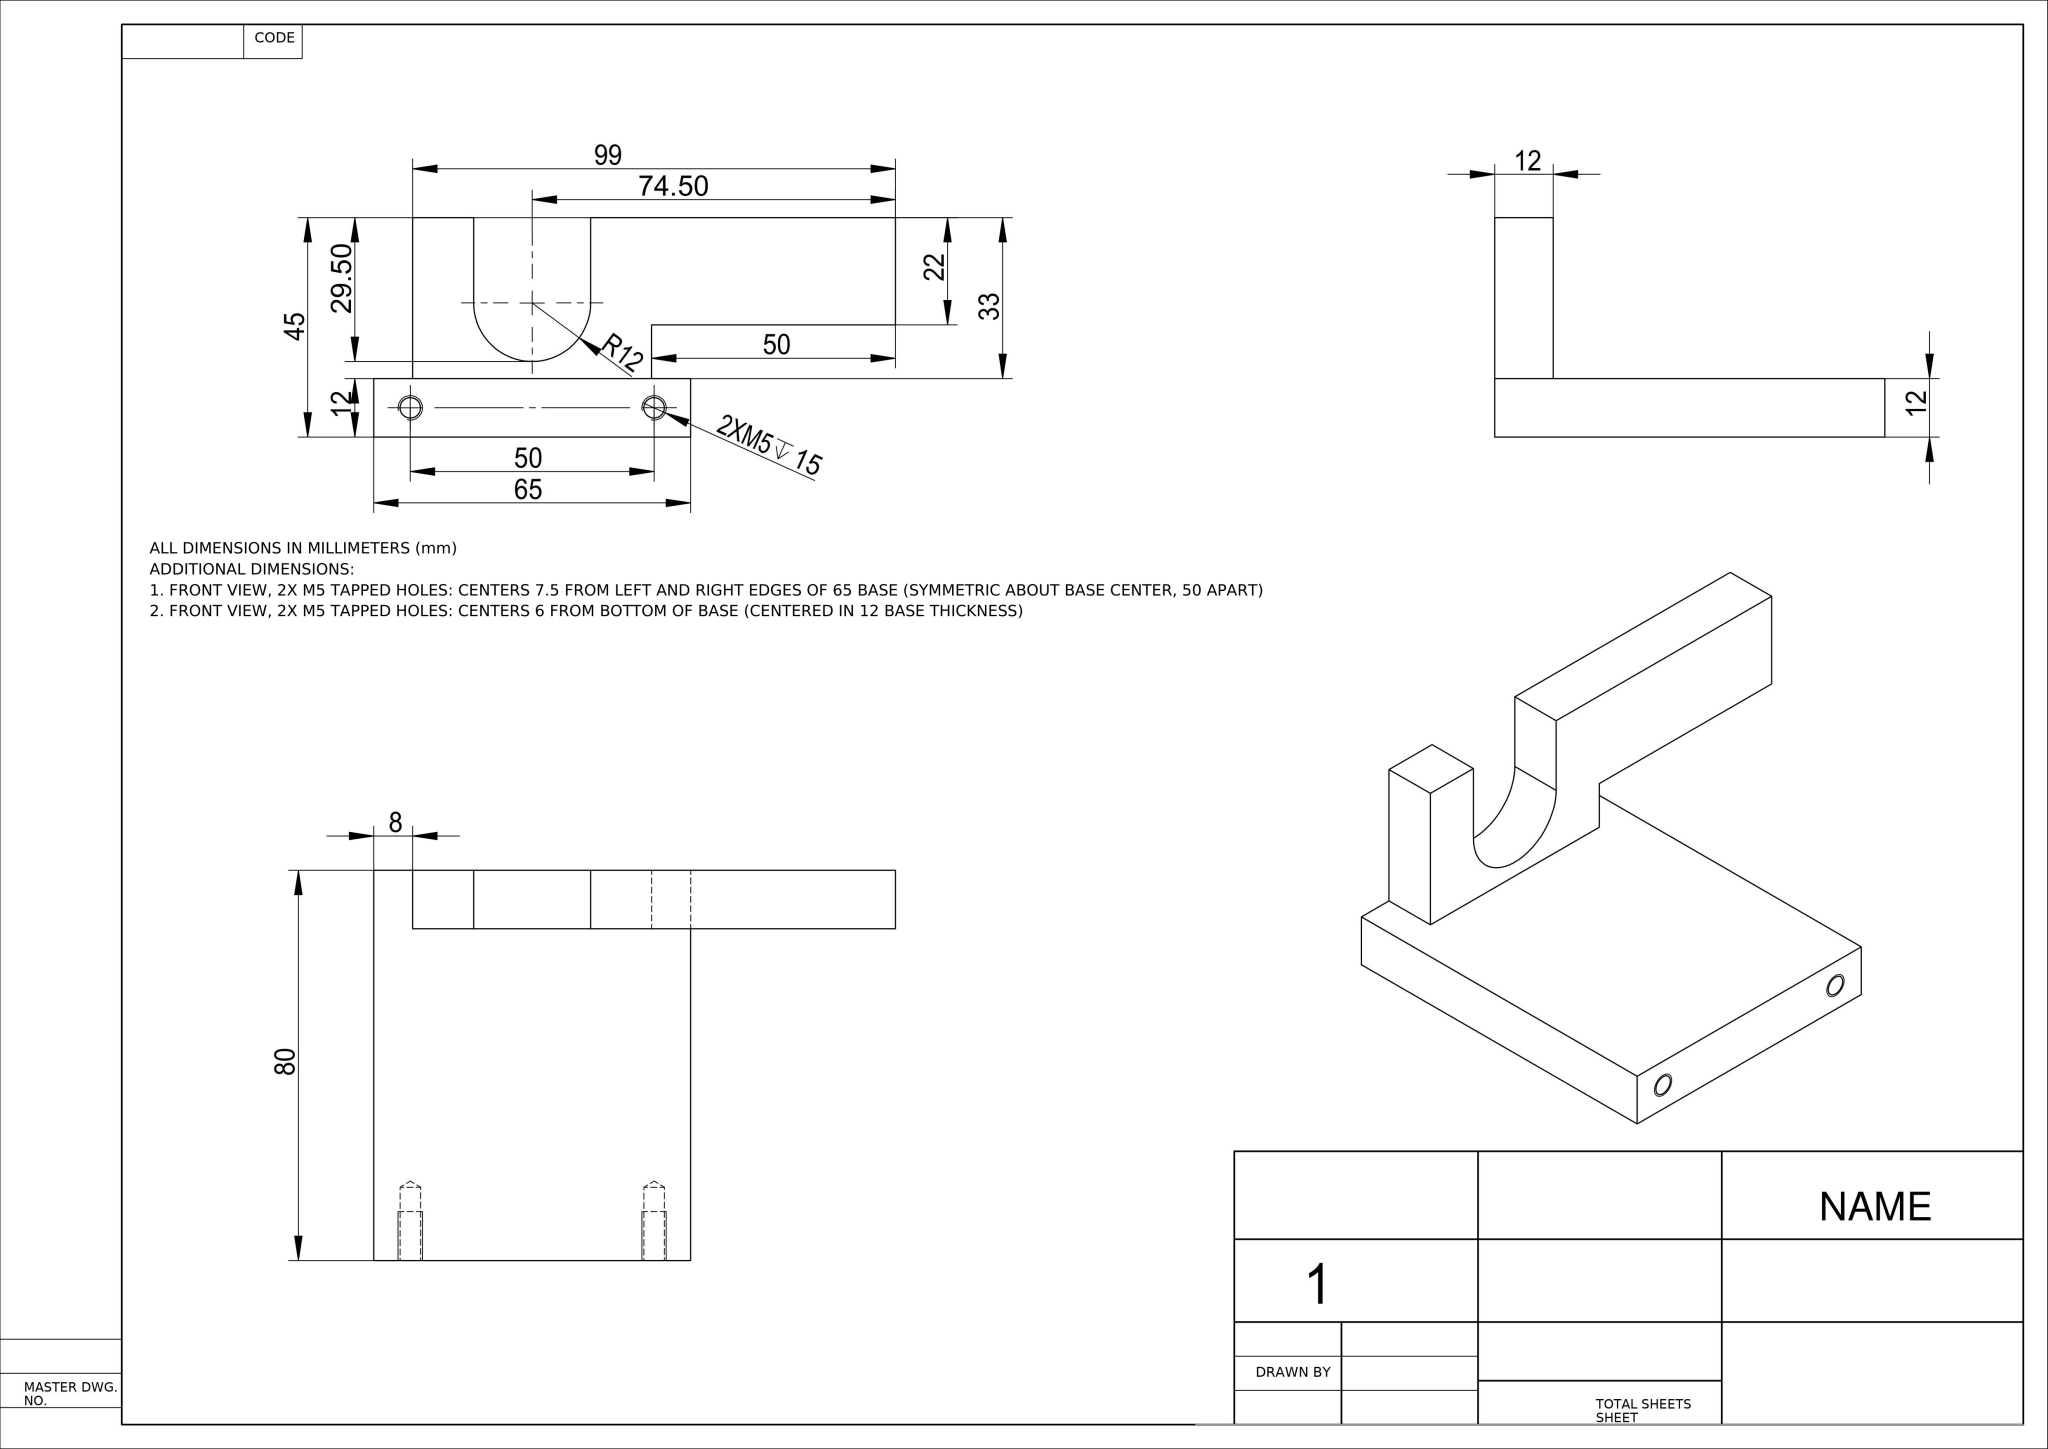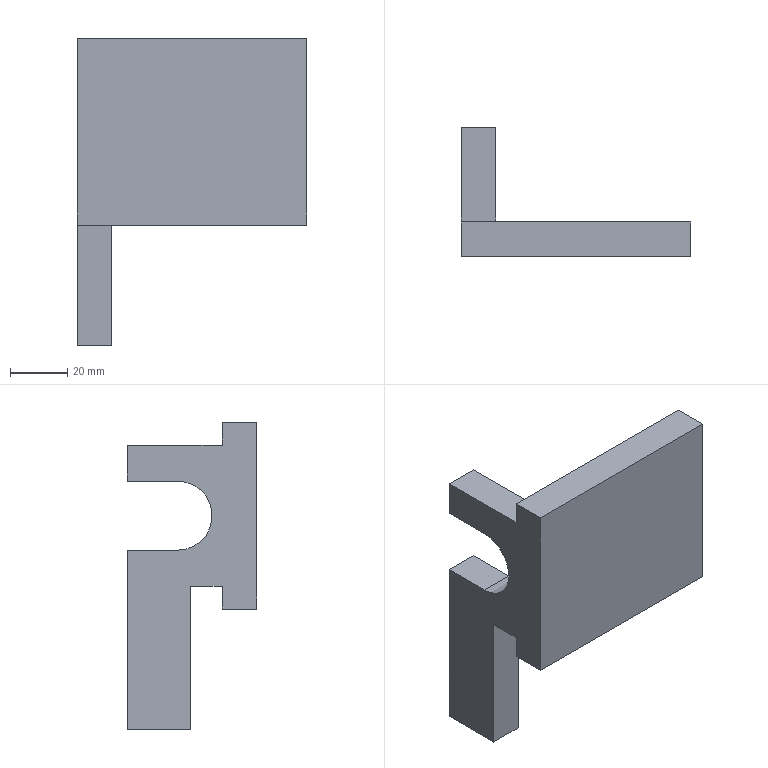Part | NX | mm | 1 solid | 24 faces | box 80 x 45 x 107 mm | volume 86822 mm3 | plane 15 | cylinder 5 | cone 4 | commonest cylinder face diameters 4.2 x4 24 x1
STEP:
#1=COLOUR_RGB('',1.,0.502,0.502);
#2=FILL_AREA_STYLE_COLOUR('',#1);
#3=FILL_AREA_STYLE('',(#2));
#4=SURFACE_STYLE_FILL_AREA(#3);
#5=SURFACE_SIDE_STYLE('',(#4));
#6=SURFACE_STYLE_USAGE(.BOTH.,#5);
#7=PRESENTATION_STYLE_ASSIGNMENT((#6));
#8=CARTESIAN_POINT('',(65.,6.,27.1));
#9=VERTEX_POINT('',#8);
#10=CARTESIAN_POINT('',(65.,6.,22.9));
#11=VERTEX_POINT('',#10);
#12=CARTESIAN_POINT('',(65.,6.,25.));
#13=DIRECTION('',(1.,0.,0.));
#14=DIRECTION('',(0.,0.,-1.));
#15=AXIS2_PLACEMENT_3D('',#12,#13,#14);
#16=CIRCLE('',#15,2.1);
#17=EDGE_CURVE('',#9,#11,#16,.T.);
#18=ORIENTED_EDGE('',*,*,#17,.F.);
#19=CARTESIAN_POINT('',(80.,6.,27.1));
#20=VERTEX_POINT('',#19);
#21=CARTESIAN_POINT('',(80.,6.,27.1));
#22=DIRECTION('',(1.,0.,0.));
#23=VECTOR('',#22,1000.);
#24=LINE('',#21,#23);
#25=EDGE_CURVE('',#9,#20,#24,.T.);
#26=ORIENTED_EDGE('',*,*,#25,.T.);
#27=CARTESIAN_POINT('',(80.,6.,22.9));
#28=VERTEX_POINT('',#27);
#29=CARTESIAN_POINT('',(80.,6.,25.));
#30=DIRECTION('',(1.,0.,0.));
#31=DIRECTION('',(0.,0.,-1.));
#32=AXIS2_PLACEMENT_3D('',#29,#30,#31);
#33=CIRCLE('',#32,2.1);
#34=EDGE_CURVE('',#20,#28,#33,.T.);
#35=ORIENTED_EDGE('',*,*,#34,.T.);
#36=CARTESIAN_POINT('',(80.,6.,22.9));
#37=DIRECTION('',(1.,0.,0.));
#38=VECTOR('',#37,1000.);
#39=LINE('',#36,#38);
#40=EDGE_CURVE('',#11,#28,#39,.T.);
#41=ORIENTED_EDGE('',*,*,#40,.F.);
#42=EDGE_LOOP('',(#18,#26,#35,#41));
#43=FACE_OUTER_BOUND('',#42,.T.);
#44=CARTESIAN_POINT('',(80.,6.,25.));
#45=DIRECTION('',(1.,0.,0.));
#46=DIRECTION('',(0.,0.,-1.));
#47=AXIS2_PLACEMENT_3D('',#44,#45,#46);
#48=CYLINDRICAL_SURFACE('',#47,2.1);
#49=ADVANCED_FACE('',(#43),#48,.F.);
#50=CARTESIAN_POINT('',(63.738,6.,25.));
#51=VERTEX_POINT('',#50);
#52=CARTESIAN_POINT('',(65.,6.,22.9));
#53=DIRECTION('',(0.515,0.,-0.8572));
#54=VECTOR('',#53,1000.);
#55=LINE('',#52,#54);
#56=EDGE_CURVE('',#51,#11,#55,.T.);
#57=ORIENTED_EDGE('',*,*,#56,.F.);
#58=CARTESIAN_POINT('',(65.,6.,27.1));
#59=DIRECTION('',(0.515,0.,0.8572));
#60=VECTOR('',#59,1000.);
#61=LINE('',#58,#60);
#62=EDGE_CURVE('',#51,#9,#61,.T.);
#63=ORIENTED_EDGE('',*,*,#62,.T.);
#64=ORIENTED_EDGE('',*,*,#17,.T.);
#65=EDGE_LOOP('',(#57,#63,#64));
#66=FACE_OUTER_BOUND('',#65,.T.);
#67=CARTESIAN_POINT('',(65.,6.,25.));
#68=DIRECTION('',(1.,0.,0.));
#69=DIRECTION('',(0.,0.,-1.));
#70=AXIS2_PLACEMENT_3D('',#67,#68,#69);
#71=CONICAL_SURFACE('',#70,2.1,1.03);
#72=ADVANCED_FACE('',(#66),#71,.F.);
#73=CARTESIAN_POINT('',(65.,6.,-22.9));
#74=VERTEX_POINT('',#73);
#75=CARTESIAN_POINT('',(65.,6.,-27.1));
#76=VERTEX_POINT('',#75);
#77=CARTESIAN_POINT('',(65.,6.,-25.));
#78=DIRECTION('',(1.,0.,0.));
#79=DIRECTION('',(0.,0.,-1.));
#80=AXIS2_PLACEMENT_3D('',#77,#78,#79);
#81=CIRCLE('',#80,2.1);
#82=EDGE_CURVE('',#74,#76,#81,.T.);
#83=ORIENTED_EDGE('',*,*,#82,.F.);
#84=CARTESIAN_POINT('',(80.,6.,-22.9));
#85=VERTEX_POINT('',#84);
#86=CARTESIAN_POINT('',(80.,6.,-22.9));
#87=DIRECTION('',(1.,0.,0.));
#88=VECTOR('',#87,1000.);
#89=LINE('',#86,#88);
#90=EDGE_CURVE('',#74,#85,#89,.T.);
#91=ORIENTED_EDGE('',*,*,#90,.T.);
#92=CARTESIAN_POINT('',(80.,6.,-27.1));
#93=VERTEX_POINT('',#92);
#94=CARTESIAN_POINT('',(80.,6.,-25.));
#95=DIRECTION('',(1.,0.,0.));
#96=DIRECTION('',(0.,0.,-1.));
#97=AXIS2_PLACEMENT_3D('',#94,#95,#96);
#98=CIRCLE('',#97,2.1);
#99=EDGE_CURVE('',#85,#93,#98,.T.);
#100=ORIENTED_EDGE('',*,*,#99,.T.);
#101=CARTESIAN_POINT('',(80.,6.,-27.1));
#102=DIRECTION('',(1.,0.,0.));
#103=VECTOR('',#102,1000.);
#104=LINE('',#101,#103);
#105=EDGE_CURVE('',#76,#93,#104,.T.);
#106=ORIENTED_EDGE('',*,*,#105,.F.);
#107=EDGE_LOOP('',(#83,#91,#100,#106));
#108=FACE_OUTER_BOUND('',#107,.T.);
#109=CARTESIAN_POINT('',(80.,6.,-25.));
#110=DIRECTION('',(1.,0.,0.));
#111=DIRECTION('',(0.,0.,-1.));
#112=AXIS2_PLACEMENT_3D('',#109,#110,#111);
#113=CYLINDRICAL_SURFACE('',#112,2.1);
#114=ADVANCED_FACE('',(#108),#113,.F.);
#115=CARTESIAN_POINT('',(63.738,6.,-25.));
#116=VERTEX_POINT('',#115);
#117=CARTESIAN_POINT('',(65.,6.,-27.1));
#118=DIRECTION('',(0.515,0.,-0.8572));
#119=VECTOR('',#118,1000.);
#120=LINE('',#117,#119);
#121=EDGE_CURVE('',#116,#76,#120,.T.);
#122=ORIENTED_EDGE('',*,*,#121,.F.);
#123=CARTESIAN_POINT('',(65.,6.,-22.9));
#124=DIRECTION('',(0.515,0.,0.8572));
#125=VECTOR('',#124,1000.);
#126=LINE('',#123,#125);
#127=EDGE_CURVE('',#116,#74,#126,.T.);
#128=ORIENTED_EDGE('',*,*,#127,.T.);
#129=ORIENTED_EDGE('',*,*,#82,.T.);
#130=EDGE_LOOP('',(#122,#128,#129));
#131=FACE_OUTER_BOUND('',#130,.T.);
#132=CARTESIAN_POINT('',(65.,6.,-25.));
#133=DIRECTION('',(1.,0.,0.));
#134=DIRECTION('',(0.,0.,-1.));
#135=AXIS2_PLACEMENT_3D('',#132,#133,#134);
#136=CONICAL_SURFACE('',#135,2.1,1.03);
#137=ADVANCED_FACE('',(#131),#136,.F.);
#138=CARTESIAN_POINT('',(12.,23.,-24.5));
#139=VERTEX_POINT('',#138);
#140=CARTESIAN_POINT('',(0.,23.,-24.5));
#141=VERTEX_POINT('',#140);
#142=CARTESIAN_POINT('',(12.,23.,-24.5));
#143=DIRECTION('',(-1.,0.,0.));
#144=VECTOR('',#143,1000.);
#145=LINE('',#142,#144);
#146=EDGE_CURVE('',#139,#141,#145,.T.);
#147=ORIENTED_EDGE('',*,*,#146,.F.);
#148=CARTESIAN_POINT('',(12.,12.,-24.5));
#149=VERTEX_POINT('',#148);
#150=CARTESIAN_POINT('',(12.,45.,-24.5));
#151=DIRECTION('',(0.,-1.,-0.));
#152=VECTOR('',#151,1000.);
#153=LINE('',#150,#152);
#154=EDGE_CURVE('',#139,#149,#153,.T.);
#155=ORIENTED_EDGE('',*,*,#154,.T.);
#156=CARTESIAN_POINT('',(0.,12.,-24.5));
#157=VERTEX_POINT('',#156);
#158=CARTESIAN_POINT('',(0.,12.,-24.5));
#159=DIRECTION('',(1.,0.,0.));
#160=VECTOR('',#159,1000.);
#161=LINE('',#158,#160);
#162=EDGE_CURVE('',#157,#149,#161,.T.);
#163=ORIENTED_EDGE('',*,*,#162,.F.);
#164=CARTESIAN_POINT('',(0.,45.,-24.5));
#165=DIRECTION('',(0.,-1.,-0.));
#166=VECTOR('',#165,1000.);
#167=LINE('',#164,#166);
#168=EDGE_CURVE('',#141,#157,#167,.T.);
#169=ORIENTED_EDGE('',*,*,#168,.F.);
#170=EDGE_LOOP('',(#147,#155,#163,#169));
#171=FACE_OUTER_BOUND('',#170,.T.);
#172=CARTESIAN_POINT('',(0.,45.,-24.5));
#173=DIRECTION('',(0.,-0.,1.));
#174=DIRECTION('',(0.,-1.,-0.));
#175=AXIS2_PLACEMENT_3D('',#172,#173,#174);
#176=PLANE('',#175);
#177=ADVANCED_FACE('',(#171),#176,.F.);
#178=CARTESIAN_POINT('',(12.,45.,-74.5));
#179=VERTEX_POINT('',#178);
#180=CARTESIAN_POINT('',(12.,45.,-12.));
#181=VERTEX_POINT('',#180);
#182=CARTESIAN_POINT('',(12.,45.,-32.5));
#183=DIRECTION('',(0.,0.,1.));
#184=VECTOR('',#183,1000.);
#185=LINE('',#182,#184);
#186=EDGE_CURVE('',#179,#181,#185,.T.);
#187=ORIENTED_EDGE('',*,*,#186,.F.);
#188=CARTESIAN_POINT('',(0.,45.,-74.5));
#189=VERTEX_POINT('',#188);
#190=CARTESIAN_POINT('',(12.,45.,-74.5));
#191=DIRECTION('',(1.,0.,0.));
#192=VECTOR('',#191,1000.);
#193=LINE('',#190,#192);
#194=EDGE_CURVE('',#189,#179,#193,.T.);
#195=ORIENTED_EDGE('',*,*,#194,.F.);
#196=CARTESIAN_POINT('',(0.,45.,-12.));
#197=VERTEX_POINT('',#196);
#198=CARTESIAN_POINT('',(0.,45.,-32.5));
#199=DIRECTION('',(0.,0.,1.));
#200=VECTOR('',#199,1000.);
#201=LINE('',#198,#200);
#202=EDGE_CURVE('',#189,#197,#201,.T.);
#203=ORIENTED_EDGE('',*,*,#202,.T.);
#204=CARTESIAN_POINT('',(80.,45.,-12.));
#205=DIRECTION('',(-1.,0.,0.));
#206=VECTOR('',#205,1000.);
#207=LINE('',#204,#206);
#208=EDGE_CURVE('',#181,#197,#207,.T.);
#209=ORIENTED_EDGE('',*,*,#208,.F.);
#210=EDGE_LOOP('',(#187,#195,#203,#209));
#211=FACE_OUTER_BOUND('',#210,.T.);
#212=CARTESIAN_POINT('',(0.,45.,-32.5));
#213=DIRECTION('',(0.,-1.,0.));
#214=DIRECTION('',(0.,0.,-1.));
#215=AXIS2_PLACEMENT_3D('',#212,#213,#214);
#216=PLANE('',#215);
#217=ADVANCED_FACE('',(#211),#216,.F.);
#218=CARTESIAN_POINT('',(0.,0.,32.5));
#219=VERTEX_POINT('',#218);
#220=CARTESIAN_POINT('',(80.,0.,32.5));
#221=VERTEX_POINT('',#220);
#222=CARTESIAN_POINT('',(0.,0.,32.5));
#223=DIRECTION('',(1.,0.,0.));
#224=VECTOR('',#223,1000.);
#225=LINE('',#222,#224);
#226=EDGE_CURVE('',#219,#221,#225,.T.);
#227=ORIENTED_EDGE('',*,*,#226,.F.);
#228=CARTESIAN_POINT('',(0.,0.,-32.5));
#229=VERTEX_POINT('',#228);
#230=CARTESIAN_POINT('',(0.,0.,-32.5));
#231=DIRECTION('',(0.,0.,1.));
#232=VECTOR('',#231,1000.);
#233=LINE('',#230,#232);
#234=EDGE_CURVE('',#229,#219,#233,.T.);
#235=ORIENTED_EDGE('',*,*,#234,.F.);
#236=CARTESIAN_POINT('',(80.,0.,-32.5));
#237=VERTEX_POINT('',#236);
#238=CARTESIAN_POINT('',(0.,0.,-32.5));
#239=DIRECTION('',(1.,0.,0.));
#240=VECTOR('',#239,1000.);
#241=LINE('',#238,#240);
#242=EDGE_CURVE('',#229,#237,#241,.T.);
#243=ORIENTED_EDGE('',*,*,#242,.T.);
#244=CARTESIAN_POINT('',(80.,0.,-32.5));
#245=DIRECTION('',(0.,0.,1.));
#246=VECTOR('',#245,1000.);
#247=LINE('',#244,#246);
#248=EDGE_CURVE('',#237,#221,#247,.T.);
#249=ORIENTED_EDGE('',*,*,#248,.T.);
#250=EDGE_LOOP('',(#227,#235,#243,#249));
#251=FACE_OUTER_BOUND('',#250,.T.);
#252=CARTESIAN_POINT('',(0.,0.,-32.5));
#253=DIRECTION('',(0.,-1.,0.));
#254=DIRECTION('',(0.,0.,-1.));
#255=AXIS2_PLACEMENT_3D('',#252,#253,#254);
#256=PLANE('',#255);
#257=ADVANCED_FACE('',(#251),#256,.T.);
#258=CARTESIAN_POINT('',(0.,12.,-32.5));
#259=VERTEX_POINT('',#258);
#260=CARTESIAN_POINT('',(0.,12.,-32.5));
#261=DIRECTION('',(0.,0.,-1.));
#262=VECTOR('',#261,1000.);
#263=LINE('',#260,#262);
#264=EDGE_CURVE('',#157,#259,#263,.T.);
#265=ORIENTED_EDGE('',*,*,#264,.T.);
#266=CARTESIAN_POINT('',(0.,45.,-32.5));
#267=DIRECTION('',(-0.,-1.,0.));
#268=VECTOR('',#267,1000.);
#269=LINE('',#266,#268);
#270=EDGE_CURVE('',#259,#229,#269,.T.);
#271=ORIENTED_EDGE('',*,*,#270,.T.);
#272=ORIENTED_EDGE('',*,*,#234,.T.);
#273=CARTESIAN_POINT('',(0.,12.,32.5));
#274=VERTEX_POINT('',#273);
#275=CARTESIAN_POINT('',(0.,45.,32.5));
#276=DIRECTION('',(-0.,-1.,0.));
#277=VECTOR('',#276,1000.);
#278=LINE('',#275,#277);
#279=EDGE_CURVE('',#274,#219,#278,.T.);
#280=ORIENTED_EDGE('',*,*,#279,.F.);
#281=CARTESIAN_POINT('',(0.,12.,24.5));
#282=VERTEX_POINT('',#281);
#283=CARTESIAN_POINT('',(0.,12.,32.5));
#284=DIRECTION('',(0.,0.,-1.));
#285=VECTOR('',#284,1000.);
#286=LINE('',#283,#285);
#287=EDGE_CURVE('',#274,#282,#286,.T.);
#288=ORIENTED_EDGE('',*,*,#287,.T.);
#289=CARTESIAN_POINT('',(0.,45.,24.5));
#290=VERTEX_POINT('',#289);
#291=CARTESIAN_POINT('',(0.,45.,24.5));
#292=DIRECTION('',(0.,1.,0.));
#293=VECTOR('',#292,1000.);
#294=LINE('',#291,#293);
#295=EDGE_CURVE('',#282,#290,#294,.T.);
#296=ORIENTED_EDGE('',*,*,#295,.T.);
#297=CARTESIAN_POINT('',(0.,45.,12.));
#298=VERTEX_POINT('',#297);
#299=CARTESIAN_POINT('',(0.,45.,-32.5));
#300=DIRECTION('',(0.,0.,1.));
#301=VECTOR('',#300,1000.);
#302=LINE('',#299,#301);
#303=EDGE_CURVE('',#298,#290,#302,.T.);
#304=ORIENTED_EDGE('',*,*,#303,.F.);
#305=CARTESIAN_POINT('',(0.,27.5,12.));
#306=VERTEX_POINT('',#305);
#307=CARTESIAN_POINT('',(0.,45.,12.));
#308=DIRECTION('',(0.,1.,0.));
#309=VECTOR('',#308,1000.);
#310=LINE('',#307,#309);
#311=EDGE_CURVE('',#306,#298,#310,.T.);
#312=ORIENTED_EDGE('',*,*,#311,.F.);
#313=CARTESIAN_POINT('',(0.,27.5,-12.));
#314=VERTEX_POINT('',#313);
#315=CARTESIAN_POINT('',(0.,27.5,0.));
#316=DIRECTION('',(-1.,0.,0.));
#317=DIRECTION('',(0.,0.,1.));
#318=AXIS2_PLACEMENT_3D('',#315,#316,#317);
#319=CIRCLE('',#318,12.);
#320=EDGE_CURVE('',#314,#306,#319,.T.);
#321=ORIENTED_EDGE('',*,*,#320,.F.);
#322=CARTESIAN_POINT('',(0.,27.5,-12.));
#323=DIRECTION('',(0.,-1.,0.));
#324=VECTOR('',#323,1000.);
#325=LINE('',#322,#324);
#326=EDGE_CURVE('',#197,#314,#325,.T.);
#327=ORIENTED_EDGE('',*,*,#326,.F.);
#328=ORIENTED_EDGE('',*,*,#202,.F.);
#329=CARTESIAN_POINT('',(0.,23.,-74.5));
#330=VERTEX_POINT('',#329);
#331=CARTESIAN_POINT('',(0.,45.,-74.5));
#332=DIRECTION('',(0.,1.,0.));
#333=VECTOR('',#332,1000.);
#334=LINE('',#331,#333);
#335=EDGE_CURVE('',#330,#189,#334,.T.);
#336=ORIENTED_EDGE('',*,*,#335,.F.);
#337=CARTESIAN_POINT('',(0.,23.,-74.5));
#338=DIRECTION('',(0.,-0.,1.));
#339=VECTOR('',#338,1000.);
#340=LINE('',#337,#339);
#341=EDGE_CURVE('',#330,#141,#340,.T.);
#342=ORIENTED_EDGE('',*,*,#341,.T.);
#343=ORIENTED_EDGE('',*,*,#168,.T.);
#344=EDGE_LOOP('',(#265,#271,#272,#280,#288,#296,#304,#312,#321,#327,#328,#336,#342,#343));
#345=FACE_OUTER_BOUND('',#344,.T.);
#346=CARTESIAN_POINT('',(0.,45.,-32.5));
#347=DIRECTION('',(-1.,0.,0.));
#348=DIRECTION('',(-0.,-1.,0.));
#349=AXIS2_PLACEMENT_3D('',#346,#347,#348);
#350=PLANE('',#349);
#351=ADVANCED_FACE('',(#345),#350,.T.);
#352=ORIENTED_EDGE('',*,*,#303,.T.);
#353=CARTESIAN_POINT('',(12.,45.,24.5));
#354=VERTEX_POINT('',#353);
#355=CARTESIAN_POINT('',(0.,45.,24.5));
#356=DIRECTION('',(1.,0.,0.));
#357=VECTOR('',#356,1000.);
#358=LINE('',#355,#357);
#359=EDGE_CURVE('',#290,#354,#358,.T.);
#360=ORIENTED_EDGE('',*,*,#359,.T.);
#361=CARTESIAN_POINT('',(12.,45.,12.));
#362=VERTEX_POINT('',#361);
#363=CARTESIAN_POINT('',(12.,45.,-32.5));
#364=DIRECTION('',(0.,0.,1.));
#365=VECTOR('',#364,1000.);
#366=LINE('',#363,#365);
#367=EDGE_CURVE('',#362,#354,#366,.T.);
#368=ORIENTED_EDGE('',*,*,#367,.F.);
#369=CARTESIAN_POINT('',(80.,45.,12.));
#370=DIRECTION('',(-1.,0.,0.));
#371=VECTOR('',#370,1000.);
#372=LINE('',#369,#371);
#373=EDGE_CURVE('',#362,#298,#372,.T.);
#374=ORIENTED_EDGE('',*,*,#373,.T.);
#375=EDGE_LOOP('',(#352,#360,#368,#374));
#376=FACE_OUTER_BOUND('',#375,.T.);
#377=CARTESIAN_POINT('',(0.,45.,-32.5));
#378=DIRECTION('',(0.,-1.,0.));
#379=DIRECTION('',(0.,0.,-1.));
#380=AXIS2_PLACEMENT_3D('',#377,#378,#379);
#381=PLANE('',#380);
#382=ADVANCED_FACE('',(#376),#381,.F.);
#383=CARTESIAN_POINT('',(12.,12.,24.5));
#384=VERTEX_POINT('',#383);
#385=CARTESIAN_POINT('',(12.,12.,-32.5));
#386=DIRECTION('',(0.,0.,1.));
#387=VECTOR('',#386,1000.);
#388=LINE('',#385,#387);
#389=EDGE_CURVE('',#149,#384,#388,.T.);
#390=ORIENTED_EDGE('',*,*,#389,.F.);
#391=ORIENTED_EDGE('',*,*,#154,.F.);
#392=CARTESIAN_POINT('',(12.,23.,-74.5));
#393=VERTEX_POINT('',#392);
#394=CARTESIAN_POINT('',(12.,23.,-74.5));
#395=DIRECTION('',(0.,-0.,1.));
#396=VECTOR('',#395,1000.);
#397=LINE('',#394,#396);
#398=EDGE_CURVE('',#393,#139,#397,.T.);
#399=ORIENTED_EDGE('',*,*,#398,.F.);
#400=CARTESIAN_POINT('',(12.,45.,-74.5));
#401=DIRECTION('',(-0.,-1.,-0.));
#402=VECTOR('',#401,1000.);
#403=LINE('',#400,#402);
#404=EDGE_CURVE('',#179,#393,#403,.T.);
#405=ORIENTED_EDGE('',*,*,#404,.F.);
#406=ORIENTED_EDGE('',*,*,#186,.T.);
#407=CARTESIAN_POINT('',(12.,27.5,-12.));
#408=VERTEX_POINT('',#407);
#409=CARTESIAN_POINT('',(12.,45.,-12.));
#410=DIRECTION('',(-0.,-1.,0.));
#411=VECTOR('',#410,1000.);
#412=LINE('',#409,#411);
#413=EDGE_CURVE('',#181,#408,#412,.T.);
#414=ORIENTED_EDGE('',*,*,#413,.T.);
#415=CARTESIAN_POINT('',(12.,27.5,12.));
#416=VERTEX_POINT('',#415);
#417=CARTESIAN_POINT('',(12.,27.5,0.));
#418=DIRECTION('',(-1.,0.,0.));
#419=DIRECTION('',(0.,-1.,0.));
#420=AXIS2_PLACEMENT_3D('',#417,#418,#419);
#421=CIRCLE('',#420,12.);
#422=EDGE_CURVE('',#408,#416,#421,.T.);
#423=ORIENTED_EDGE('',*,*,#422,.T.);
#424=CARTESIAN_POINT('',(12.,45.,12.));
#425=DIRECTION('',(0.,1.,0.));
#426=VECTOR('',#425,1000.);
#427=LINE('',#424,#426);
#428=EDGE_CURVE('',#416,#362,#427,.T.);
#429=ORIENTED_EDGE('',*,*,#428,.T.);
#430=ORIENTED_EDGE('',*,*,#367,.T.);
#431=CARTESIAN_POINT('',(12.,45.,24.5));
#432=DIRECTION('',(0.,1.,0.));
#433=VECTOR('',#432,1000.);
#434=LINE('',#431,#433);
#435=EDGE_CURVE('',#384,#354,#434,.T.);
#436=ORIENTED_EDGE('',*,*,#435,.F.);
#437=EDGE_LOOP('',(#390,#391,#399,#405,#406,#414,#423,#429,#430,#436));
#438=FACE_OUTER_BOUND('',#437,.T.);
#439=CARTESIAN_POINT('',(12.,45.,-32.5));
#440=DIRECTION('',(-1.,0.,0.));
#441=DIRECTION('',(-0.,-1.,0.));
#442=AXIS2_PLACEMENT_3D('',#439,#440,#441);
#443=PLANE('',#442);
#444=ADVANCED_FACE('',(#438),#443,.F.);
#445=CARTESIAN_POINT('',(80.,12.,32.5));
#446=VERTEX_POINT('',#445);
#447=CARTESIAN_POINT('',(0.,12.,32.5));
#448=DIRECTION('',(1.,0.,0.));
#449=VECTOR('',#448,1000.);
#450=LINE('',#447,#449);
#451=EDGE_CURVE('',#274,#446,#450,.T.);
#452=ORIENTED_EDGE('',*,*,#451,.T.);
#453=CARTESIAN_POINT('',(80.,12.,-32.5));
#454=VERTEX_POINT('',#453);
#455=CARTESIAN_POINT('',(80.,12.,-32.5));
#456=DIRECTION('',(0.,0.,1.));
#457=VECTOR('',#456,1000.);
#458=LINE('',#455,#457);
#459=EDGE_CURVE('',#454,#446,#458,.T.);
#460=ORIENTED_EDGE('',*,*,#459,.F.);
#461=CARTESIAN_POINT('',(0.,12.,-32.5));
#462=DIRECTION('',(1.,0.,0.));
#463=VECTOR('',#462,1000.);
#464=LINE('',#461,#463);
#465=EDGE_CURVE('',#259,#454,#464,.T.);
#466=ORIENTED_EDGE('',*,*,#465,.F.);
#467=ORIENTED_EDGE('',*,*,#264,.F.);
#468=ORIENTED_EDGE('',*,*,#162,.T.);
#469=ORIENTED_EDGE('',*,*,#389,.T.);
#470=CARTESIAN_POINT('',(0.,12.,24.5));
#471=DIRECTION('',(1.,0.,0.));
#472=VECTOR('',#471,1000.);
#473=LINE('',#470,#472);
#474=EDGE_CURVE('',#282,#384,#473,.T.);
#475=ORIENTED_EDGE('',*,*,#474,.F.);
#476=ORIENTED_EDGE('',*,*,#287,.F.);
#477=EDGE_LOOP('',(#452,#460,#466,#467,#468,#469,#475,#476));
#478=FACE_OUTER_BOUND('',#477,.T.);
#479=CARTESIAN_POINT('',(0.,12.,-32.5));
#480=DIRECTION('',(0.,-1.,0.));
#481=DIRECTION('',(0.,0.,-1.));
#482=AXIS2_PLACEMENT_3D('',#479,#480,#481);
#483=PLANE('',#482);
#484=ADVANCED_FACE('',(#478),#483,.F.);
#485=CARTESIAN_POINT('',(80.,6.,25.));
#486=DIRECTION('',(1.,0.,0.));
#487=DIRECTION('',(0.,0.,-1.));
#488=AXIS2_PLACEMENT_3D('',#485,#486,#487);
#489=CIRCLE('',#488,2.1);
#490=EDGE_CURVE('',#28,#20,#489,.T.);
#491=ORIENTED_EDGE('',*,*,#490,.F.);
#492=ORIENTED_EDGE('',*,*,#34,.F.);
#493=EDGE_LOOP('',(#491,#492));
#494=FACE_BOUND('',#493,.T.);
#495=CARTESIAN_POINT('',(80.,6.,-25.));
#496=DIRECTION('',(1.,0.,0.));
#497=DIRECTION('',(0.,0.,-1.));
#498=AXIS2_PLACEMENT_3D('',#495,#496,#497);
#499=CIRCLE('',#498,2.1);
#500=EDGE_CURVE('',#93,#85,#499,.T.);
#501=ORIENTED_EDGE('',*,*,#500,.F.);
#502=ORIENTED_EDGE('',*,*,#99,.F.);
#503=EDGE_LOOP('',(#501,#502));
#504=FACE_BOUND('',#503,.T.);
#505=CARTESIAN_POINT('',(80.,12.,32.5));
#506=DIRECTION('',(0.,-1.,0.));
#507=VECTOR('',#506,1000.);
#508=LINE('',#505,#507);
#509=EDGE_CURVE('',#446,#221,#508,.T.);
#510=ORIENTED_EDGE('',*,*,#509,.T.);
#511=ORIENTED_EDGE('',*,*,#248,.F.);
#512=CARTESIAN_POINT('',(80.,12.,-32.5));
#513=DIRECTION('',(0.,-1.,0.));
#514=VECTOR('',#513,1000.);
#515=LINE('',#512,#514);
#516=EDGE_CURVE('',#454,#237,#515,.T.);
#517=ORIENTED_EDGE('',*,*,#516,.F.);
#518=ORIENTED_EDGE('',*,*,#459,.T.);
#519=EDGE_LOOP('',(#510,#511,#517,#518));
#520=FACE_OUTER_BOUND('',#519,.T.);
#521=CARTESIAN_POINT('',(80.,12.,-32.5));
#522=DIRECTION('',(-1.,0.,0.));
#523=DIRECTION('',(0.,0.,1.));
#524=AXIS2_PLACEMENT_3D('',#521,#522,#523);
#525=PLANE('',#524);
#526=ADVANCED_FACE('',(#494,#504,#520),#525,.F.);
#527=ORIENTED_EDGE('',*,*,#270,.F.);
#528=ORIENTED_EDGE('',*,*,#465,.T.);
#529=ORIENTED_EDGE('',*,*,#516,.T.);
#530=ORIENTED_EDGE('',*,*,#242,.F.);
#531=EDGE_LOOP('',(#527,#528,#529,#530));
#532=FACE_OUTER_BOUND('',#531,.T.);
#533=CARTESIAN_POINT('',(0.,0.,-32.5));
#534=DIRECTION('',(0.,0.,-1.));
#535=DIRECTION('',(-1.,0.,0.));
#536=AXIS2_PLACEMENT_3D('',#533,#534,#535);
#537=PLANE('',#536);
#538=ADVANCED_FACE('',(#532),#537,.T.);
#539=ORIENTED_EDGE('',*,*,#451,.F.);
#540=ORIENTED_EDGE('',*,*,#279,.T.);
#541=ORIENTED_EDGE('',*,*,#226,.T.);
#542=ORIENTED_EDGE('',*,*,#509,.F.);
#543=EDGE_LOOP('',(#539,#540,#541,#542));
#544=FACE_OUTER_BOUND('',#543,.T.);
#545=CARTESIAN_POINT('',(0.,0.,32.5));
#546=DIRECTION('',(0.,0.,-1.));
#547=DIRECTION('',(-1.,0.,0.));
#548=AXIS2_PLACEMENT_3D('',#545,#546,#547);
#549=PLANE('',#548);
#550=ADVANCED_FACE('',(#544),#549,.F.);
#551=CARTESIAN_POINT('',(80.,27.5,-12.));
#552=DIRECTION('',(-1.,0.,0.));
#553=VECTOR('',#552,1000.);
#554=LINE('',#551,#553);
#555=EDGE_CURVE('',#408,#314,#554,.T.);
#556=ORIENTED_EDGE('',*,*,#555,.T.);
#557=ORIENTED_EDGE('',*,*,#320,.T.);
#558=CARTESIAN_POINT('',(80.,27.5,12.));
#559=DIRECTION('',(-1.,0.,0.));
#560=VECTOR('',#559,1000.);
#561=LINE('',#558,#560);
#562=EDGE_CURVE('',#416,#306,#561,.T.);
#563=ORIENTED_EDGE('',*,*,#562,.F.);
#564=ORIENTED_EDGE('',*,*,#422,.F.);
#565=EDGE_LOOP('',(#556,#557,#563,#564));
#566=FACE_OUTER_BOUND('',#565,.T.);
#567=CARTESIAN_POINT('',(80.,27.5,0.));
#568=DIRECTION('',(-1.,0.,0.));
#569=DIRECTION('',(0.,0.,1.));
#570=AXIS2_PLACEMENT_3D('',#567,#568,#569);
#571=CYLINDRICAL_SURFACE('',#570,12.);
#572=ADVANCED_FACE('',(#566),#571,.F.);
#573=ORIENTED_EDGE('',*,*,#208,.T.);
#574=ORIENTED_EDGE('',*,*,#326,.T.);
#575=ORIENTED_EDGE('',*,*,#555,.F.);
#576=ORIENTED_EDGE('',*,*,#413,.F.);
#577=EDGE_LOOP('',(#573,#574,#575,#576));
#578=FACE_OUTER_BOUND('',#577,.T.);
#579=CARTESIAN_POINT('',(80.,27.5,-12.));
#580=DIRECTION('',(0.,-0.,-1.));
#581=DIRECTION('',(0.,1.,-0.));
#582=AXIS2_PLACEMENT_3D('',#579,#580,#581);
#583=PLANE('',#582);
#584=ADVANCED_FACE('',(#578),#583,.F.);
#585=ORIENTED_EDGE('',*,*,#562,.T.);
#586=ORIENTED_EDGE('',*,*,#311,.T.);
#587=ORIENTED_EDGE('',*,*,#373,.F.);
#588=ORIENTED_EDGE('',*,*,#428,.F.);
#589=EDGE_LOOP('',(#585,#586,#587,#588));
#590=FACE_OUTER_BOUND('',#589,.T.);
#591=CARTESIAN_POINT('',(80.,45.,12.));
#592=DIRECTION('',(0.,-0.,1.));
#593=DIRECTION('',(0.,-1.,-0.));
#594=AXIS2_PLACEMENT_3D('',#591,#592,#593);
#595=PLANE('',#594);
#596=ADVANCED_FACE('',(#590),#595,.F.);
#597=ORIENTED_EDGE('',*,*,#435,.T.);
#598=ORIENTED_EDGE('',*,*,#359,.F.);
#599=ORIENTED_EDGE('',*,*,#295,.F.);
#600=ORIENTED_EDGE('',*,*,#474,.T.);
#601=EDGE_LOOP('',(#597,#598,#599,#600));
#602=FACE_OUTER_BOUND('',#601,.T.);
#603=CARTESIAN_POINT('',(0.,45.,24.5));
#604=DIRECTION('',(0.,0.,-1.));
#605=DIRECTION('',(0.,1.,0.));
#606=AXIS2_PLACEMENT_3D('',#603,#604,#605);
#607=PLANE('',#606);
#608=ADVANCED_FACE('',(#602),#607,.F.);
#609=ORIENTED_EDGE('',*,*,#146,.T.);
#610=ORIENTED_EDGE('',*,*,#341,.F.);
#611=CARTESIAN_POINT('',(12.,23.,-74.5));
#612=DIRECTION('',(-1.,0.,0.));
#613=VECTOR('',#612,1000.);
#614=LINE('',#611,#613);
#615=EDGE_CURVE('',#393,#330,#614,.T.);
#616=ORIENTED_EDGE('',*,*,#615,.F.);
#617=ORIENTED_EDGE('',*,*,#398,.T.);
#618=EDGE_LOOP('',(#609,#610,#616,#617));
#619=FACE_OUTER_BOUND('',#618,.T.);
#620=CARTESIAN_POINT('',(12.,23.,-74.5));
#621=DIRECTION('',(0.,1.,0.));
#622=DIRECTION('',(0.,-0.,1.));
#623=AXIS2_PLACEMENT_3D('',#620,#621,#622);
#624=PLANE('',#623);
#625=ADVANCED_FACE('',(#619),#624,.F.);
#626=ORIENTED_EDGE('',*,*,#404,.T.);
#627=ORIENTED_EDGE('',*,*,#615,.T.);
#628=ORIENTED_EDGE('',*,*,#335,.T.);
#629=ORIENTED_EDGE('',*,*,#194,.T.);
#630=EDGE_LOOP('',(#626,#627,#628,#629));
#631=FACE_OUTER_BOUND('',#630,.T.);
#632=CARTESIAN_POINT('',(0.,0.,-74.5));
#633=DIRECTION('',(0.,0.,-1.));
#634=DIRECTION('',(0.,1.,0.));
#635=AXIS2_PLACEMENT_3D('',#632,#633,#634);
#636=PLANE('',#635);
#637=ADVANCED_FACE('',(#631),#636,.T.);
#638=ORIENTED_EDGE('',*,*,#127,.F.);
#639=ORIENTED_EDGE('',*,*,#121,.T.);
#640=CARTESIAN_POINT('',(65.,6.,-25.));
#641=DIRECTION('',(1.,0.,0.));
#642=DIRECTION('',(0.,0.,-1.));
#643=AXIS2_PLACEMENT_3D('',#640,#641,#642);
#644=CIRCLE('',#643,2.1);
#645=EDGE_CURVE('',#76,#74,#644,.T.);
#646=ORIENTED_EDGE('',*,*,#645,.T.);
#647=EDGE_LOOP('',(#638,#639,#646));
#648=FACE_OUTER_BOUND('',#647,.T.);
#649=CARTESIAN_POINT('',(65.,6.,-25.));
#650=DIRECTION('',(1.,0.,0.));
#651=DIRECTION('',(0.,0.,-1.));
#652=AXIS2_PLACEMENT_3D('',#649,#650,#651);
#653=CONICAL_SURFACE('',#652,2.1,1.03);
#654=ADVANCED_FACE('',(#648),#653,.F.);
#655=ORIENTED_EDGE('',*,*,#90,.F.);
#656=ORIENTED_EDGE('',*,*,#645,.F.);
#657=ORIENTED_EDGE('',*,*,#105,.T.);
#658=ORIENTED_EDGE('',*,*,#500,.T.);
#659=EDGE_LOOP('',(#655,#656,#657,#658));
#660=FACE_OUTER_BOUND('',#659,.T.);
#661=CARTESIAN_POINT('',(80.,6.,-25.));
#662=DIRECTION('',(1.,0.,0.));
#663=DIRECTION('',(0.,0.,-1.));
#664=AXIS2_PLACEMENT_3D('',#661,#662,#663);
#665=CYLINDRICAL_SURFACE('',#664,2.1);
#666=ADVANCED_FACE('',(#660),#665,.F.);
#667=ORIENTED_EDGE('',*,*,#62,.F.);
#668=ORIENTED_EDGE('',*,*,#56,.T.);
#669=CARTESIAN_POINT('',(65.,6.,25.));
#670=DIRECTION('',(1.,0.,0.));
#671=DIRECTION('',(0.,0.,-1.));
#672=AXIS2_PLACEMENT_3D('',#669,#670,#671);
#673=CIRCLE('',#672,2.1);
#674=EDGE_CURVE('',#11,#9,#673,.T.);
#675=ORIENTED_EDGE('',*,*,#674,.T.);
#676=EDGE_LOOP('',(#667,#668,#675));
#677=FACE_OUTER_BOUND('',#676,.T.);
#678=CARTESIAN_POINT('',(65.,6.,25.));
#679=DIRECTION('',(1.,0.,0.));
#680=DIRECTION('',(0.,0.,-1.));
#681=AXIS2_PLACEMENT_3D('',#678,#679,#680);
#682=CONICAL_SURFACE('',#681,2.1,1.03);
#683=ADVANCED_FACE('',(#677),#682,.F.);
#684=ORIENTED_EDGE('',*,*,#25,.F.);
#685=ORIENTED_EDGE('',*,*,#674,.F.);
#686=ORIENTED_EDGE('',*,*,#40,.T.);
#687=ORIENTED_EDGE('',*,*,#490,.T.);
#688=EDGE_LOOP('',(#684,#685,#686,#687));
#689=FACE_OUTER_BOUND('',#688,.T.);
#690=CARTESIAN_POINT('',(80.,6.,25.));
#691=DIRECTION('',(1.,0.,0.));
#692=DIRECTION('',(0.,0.,-1.));
#693=AXIS2_PLACEMENT_3D('',#690,#691,#692);
#694=CYLINDRICAL_SURFACE('',#693,2.1);
#695=ADVANCED_FACE('',(#689),#694,.F.);
#696=CLOSED_SHELL('',(#49,#72,#114,#137,#177,#217,#257,#351,#382,#444,#484,#526,#538,#550,#572,#584,#596,#608,#625,#637,#654,#666,#683,#695));
#697=MANIFOLD_SOLID_BREP('',#696);
#698=STYLED_ITEM('',(#7),#697);
#699=PRESENTATION_LAYER_ASSIGNMENT('','',(#698));
#700=COLOUR_RGB('',1.,0.502,0.502);
#701=FILL_AREA_STYLE_COLOUR('',#700);
#702=FILL_AREA_STYLE('',(#701));
#703=SURFACE_STYLE_FILL_AREA(#702);
#704=SURFACE_SIDE_STYLE('',(#703));
#705=SURFACE_STYLE_USAGE(.BOTH.,#704);
#706=PRESENTATION_STYLE_ASSIGNMENT((#705));
#707=STYLED_ITEM('',(#706),#49);
#708=PRESENTATION_LAYER_ASSIGNMENT('','',(#707));
#709=COLOUR_RGB('',1.,0.502,0.502);
#710=FILL_AREA_STYLE_COLOUR('',#709);
#711=FILL_AREA_STYLE('',(#710));
#712=SURFACE_STYLE_FILL_AREA(#711);
#713=SURFACE_SIDE_STYLE('',(#712));
#714=SURFACE_STYLE_USAGE(.BOTH.,#713);
#715=PRESENTATION_STYLE_ASSIGNMENT((#714));
#716=STYLED_ITEM('',(#715),#695);
#717=(LENGTH_UNIT()NAMED_UNIT(*)SI_UNIT(.MILLI.,.METRE.));
#718=UNCERTAINTY_MEASURE_WITH_UNIT(LENGTH_MEASURE(0.00001),#717,'','');
#719=(NAMED_UNIT(*)PLANE_ANGLE_UNIT()SI_UNIT($,.RADIAN.));
#720=(NAMED_UNIT(*)SI_UNIT($,.STERADIAN.)SOLID_ANGLE_UNIT());
#721=(GEOMETRIC_REPRESENTATION_CONTEXT(3)GLOBAL_UNCERTAINTY_ASSIGNED_CONTEXT((#718))GLOBAL_UNIT_ASSIGNED_CONTEXT((#717,#719,#720))REPRESENTATION_CONTEXT('',''));
#722=MECHANICAL_DESIGN_GEOMETRIC_PRESENTATION_REPRESENTATION('',(#716),#721);
#723=COLOUR_RGB('',1.,0.502,0.502);
#724=FILL_AREA_STYLE_COLOUR('',#723);
#725=FILL_AREA_STYLE('',(#724));
#726=SURFACE_STYLE_FILL_AREA(#725);
#727=SURFACE_SIDE_STYLE('',(#726));
#728=SURFACE_STYLE_USAGE(.BOTH.,#727);
#729=PRESENTATION_STYLE_ASSIGNMENT((#728));
#730=STYLED_ITEM('',(#729),#114);
#731=(LENGTH_UNIT()NAMED_UNIT(*)SI_UNIT(.MILLI.,.METRE.));
#732=UNCERTAINTY_MEASURE_WITH_UNIT(LENGTH_MEASURE(0.00001),#731,'','');
#733=(NAMED_UNIT(*)PLANE_ANGLE_UNIT()SI_UNIT($,.RADIAN.));
#734=(NAMED_UNIT(*)SI_UNIT($,.STERADIAN.)SOLID_ANGLE_UNIT());
#735=(GEOMETRIC_REPRESENTATION_CONTEXT(3)GLOBAL_UNCERTAINTY_ASSIGNED_CONTEXT((#732))GLOBAL_UNIT_ASSIGNED_CONTEXT((#731,#733,#734))REPRESENTATION_CONTEXT('',''));
#736=MECHANICAL_DESIGN_GEOMETRIC_PRESENTATION_REPRESENTATION('',(#730),#735);
#737=COLOUR_RGB('',1.,0.502,0.502);
#738=FILL_AREA_STYLE_COLOUR('',#737);
#739=FILL_AREA_STYLE('',(#738));
#740=SURFACE_STYLE_FILL_AREA(#739);
#741=SURFACE_SIDE_STYLE('',(#740));
#742=SURFACE_STYLE_USAGE(.BOTH.,#741);
#743=PRESENTATION_STYLE_ASSIGNMENT((#742));
#744=CARTESIAN_POINT('',(0.,0.,0.));
#745=DIRECTION('',(0.,0.,1.));
#746=DIRECTION('',(1.,0.,0.));
#747=AXIS2_PLACEMENT_3D('',#744,#745,#746);
#748=(LENGTH_UNIT()NAMED_UNIT(*)SI_UNIT(.MILLI.,.METRE.));
#749=UNCERTAINTY_MEASURE_WITH_UNIT(LENGTH_MEASURE(0.00001),#748,'','');
#750=(NAMED_UNIT(*)PLANE_ANGLE_UNIT()SI_UNIT($,.RADIAN.));
#751=(NAMED_UNIT(*)SI_UNIT($,.STERADIAN.)SOLID_ANGLE_UNIT());
#752=(GEOMETRIC_REPRESENTATION_CONTEXT(3)GLOBAL_UNCERTAINTY_ASSIGNED_CONTEXT((#749))GLOBAL_UNIT_ASSIGNED_CONTEXT((#748,#750,#751))REPRESENTATION_CONTEXT('',''));
#753=ADVANCED_BREP_SHAPE_REPRESENTATION('',(#697,#747),#752);
#754=STYLED_ITEM('',(#743),#753);
#755=(LENGTH_UNIT()NAMED_UNIT(*)SI_UNIT(.MILLI.,.METRE.));
#756=UNCERTAINTY_MEASURE_WITH_UNIT(LENGTH_MEASURE(0.00001),#755,'','');
#757=(NAMED_UNIT(*)PLANE_ANGLE_UNIT()SI_UNIT($,.RADIAN.));
#758=(NAMED_UNIT(*)SI_UNIT($,.STERADIAN.)SOLID_ANGLE_UNIT());
#759=(GEOMETRIC_REPRESENTATION_CONTEXT(3)GLOBAL_UNCERTAINTY_ASSIGNED_CONTEXT((#756))GLOBAL_UNIT_ASSIGNED_CONTEXT((#755,#757,#758))REPRESENTATION_CONTEXT('',''));
#760=MECHANICAL_DESIGN_GEOMETRIC_PRESENTATION_REPRESENTATION('',(#754),#759);
#761=PRESENTATION_LAYER_ASSIGNMENT('','',(#730));
#762=COLOUR_RGB('',1.,0.502,0.502);
#763=FILL_AREA_STYLE_COLOUR('',#762);
#764=FILL_AREA_STYLE('',(#763));
#765=SURFACE_STYLE_FILL_AREA(#764);
#766=SURFACE_SIDE_STYLE('',(#765));
#767=SURFACE_STYLE_USAGE(.BOTH.,#766);
#768=PRESENTATION_STYLE_ASSIGNMENT((#767));
#769=STYLED_ITEM('',(#768),#666);
#770=PRESENTATION_LAYER_ASSIGNMENT('','',(#769));
#771=(LENGTH_UNIT()NAMED_UNIT(*)SI_UNIT(.MILLI.,.METRE.));
#772=UNCERTAINTY_MEASURE_WITH_UNIT(LENGTH_MEASURE(0.00001),#771,'','');
#773=(NAMED_UNIT(*)PLANE_ANGLE_UNIT()SI_UNIT($,.RADIAN.));
#774=(NAMED_UNIT(*)SI_UNIT($,.STERADIAN.)SOLID_ANGLE_UNIT());
#775=(GEOMETRIC_REPRESENTATION_CONTEXT(3)GLOBAL_UNCERTAINTY_ASSIGNED_CONTEXT((#772))GLOBAL_UNIT_ASSIGNED_CONTEXT((#771,#773,#774))REPRESENTATION_CONTEXT('',''));
#776=MECHANICAL_DESIGN_GEOMETRIC_PRESENTATION_REPRESENTATION('',(#698),#775);
#777=PRESENTATION_LAYER_ASSIGNMENT('','',(#716));
#778=PRESENTATION_LAYER_ASSIGNMENT('','',(#754));
#779=(LENGTH_UNIT()NAMED_UNIT(*)SI_UNIT(.MILLI.,.METRE.));
#780=UNCERTAINTY_MEASURE_WITH_UNIT(LENGTH_MEASURE(0.00001),#779,'','');
#781=(NAMED_UNIT(*)PLANE_ANGLE_UNIT()SI_UNIT($,.RADIAN.));
#782=(NAMED_UNIT(*)SI_UNIT($,.STERADIAN.)SOLID_ANGLE_UNIT());
#783=(GEOMETRIC_REPRESENTATION_CONTEXT(3)GLOBAL_UNCERTAINTY_ASSIGNED_CONTEXT((#780))GLOBAL_UNIT_ASSIGNED_CONTEXT((#779,#781,#782))REPRESENTATION_CONTEXT('',''));
#784=MECHANICAL_DESIGN_GEOMETRIC_PRESENTATION_REPRESENTATION('',(#707),#783);
#785=(LENGTH_UNIT()NAMED_UNIT(*)SI_UNIT(.MILLI.,.METRE.));
#786=UNCERTAINTY_MEASURE_WITH_UNIT(LENGTH_MEASURE(0.00001),#785,'','');
#787=(NAMED_UNIT(*)PLANE_ANGLE_UNIT()SI_UNIT($,.RADIAN.));
#788=(NAMED_UNIT(*)SI_UNIT($,.STERADIAN.)SOLID_ANGLE_UNIT());
#789=(GEOMETRIC_REPRESENTATION_CONTEXT(3)GLOBAL_UNCERTAINTY_ASSIGNED_CONTEXT((#786))GLOBAL_UNIT_ASSIGNED_CONTEXT((#785,#787,#788))REPRESENTATION_CONTEXT('',''));
#790=MECHANICAL_DESIGN_GEOMETRIC_PRESENTATION_REPRESENTATION('',(#769),#789);